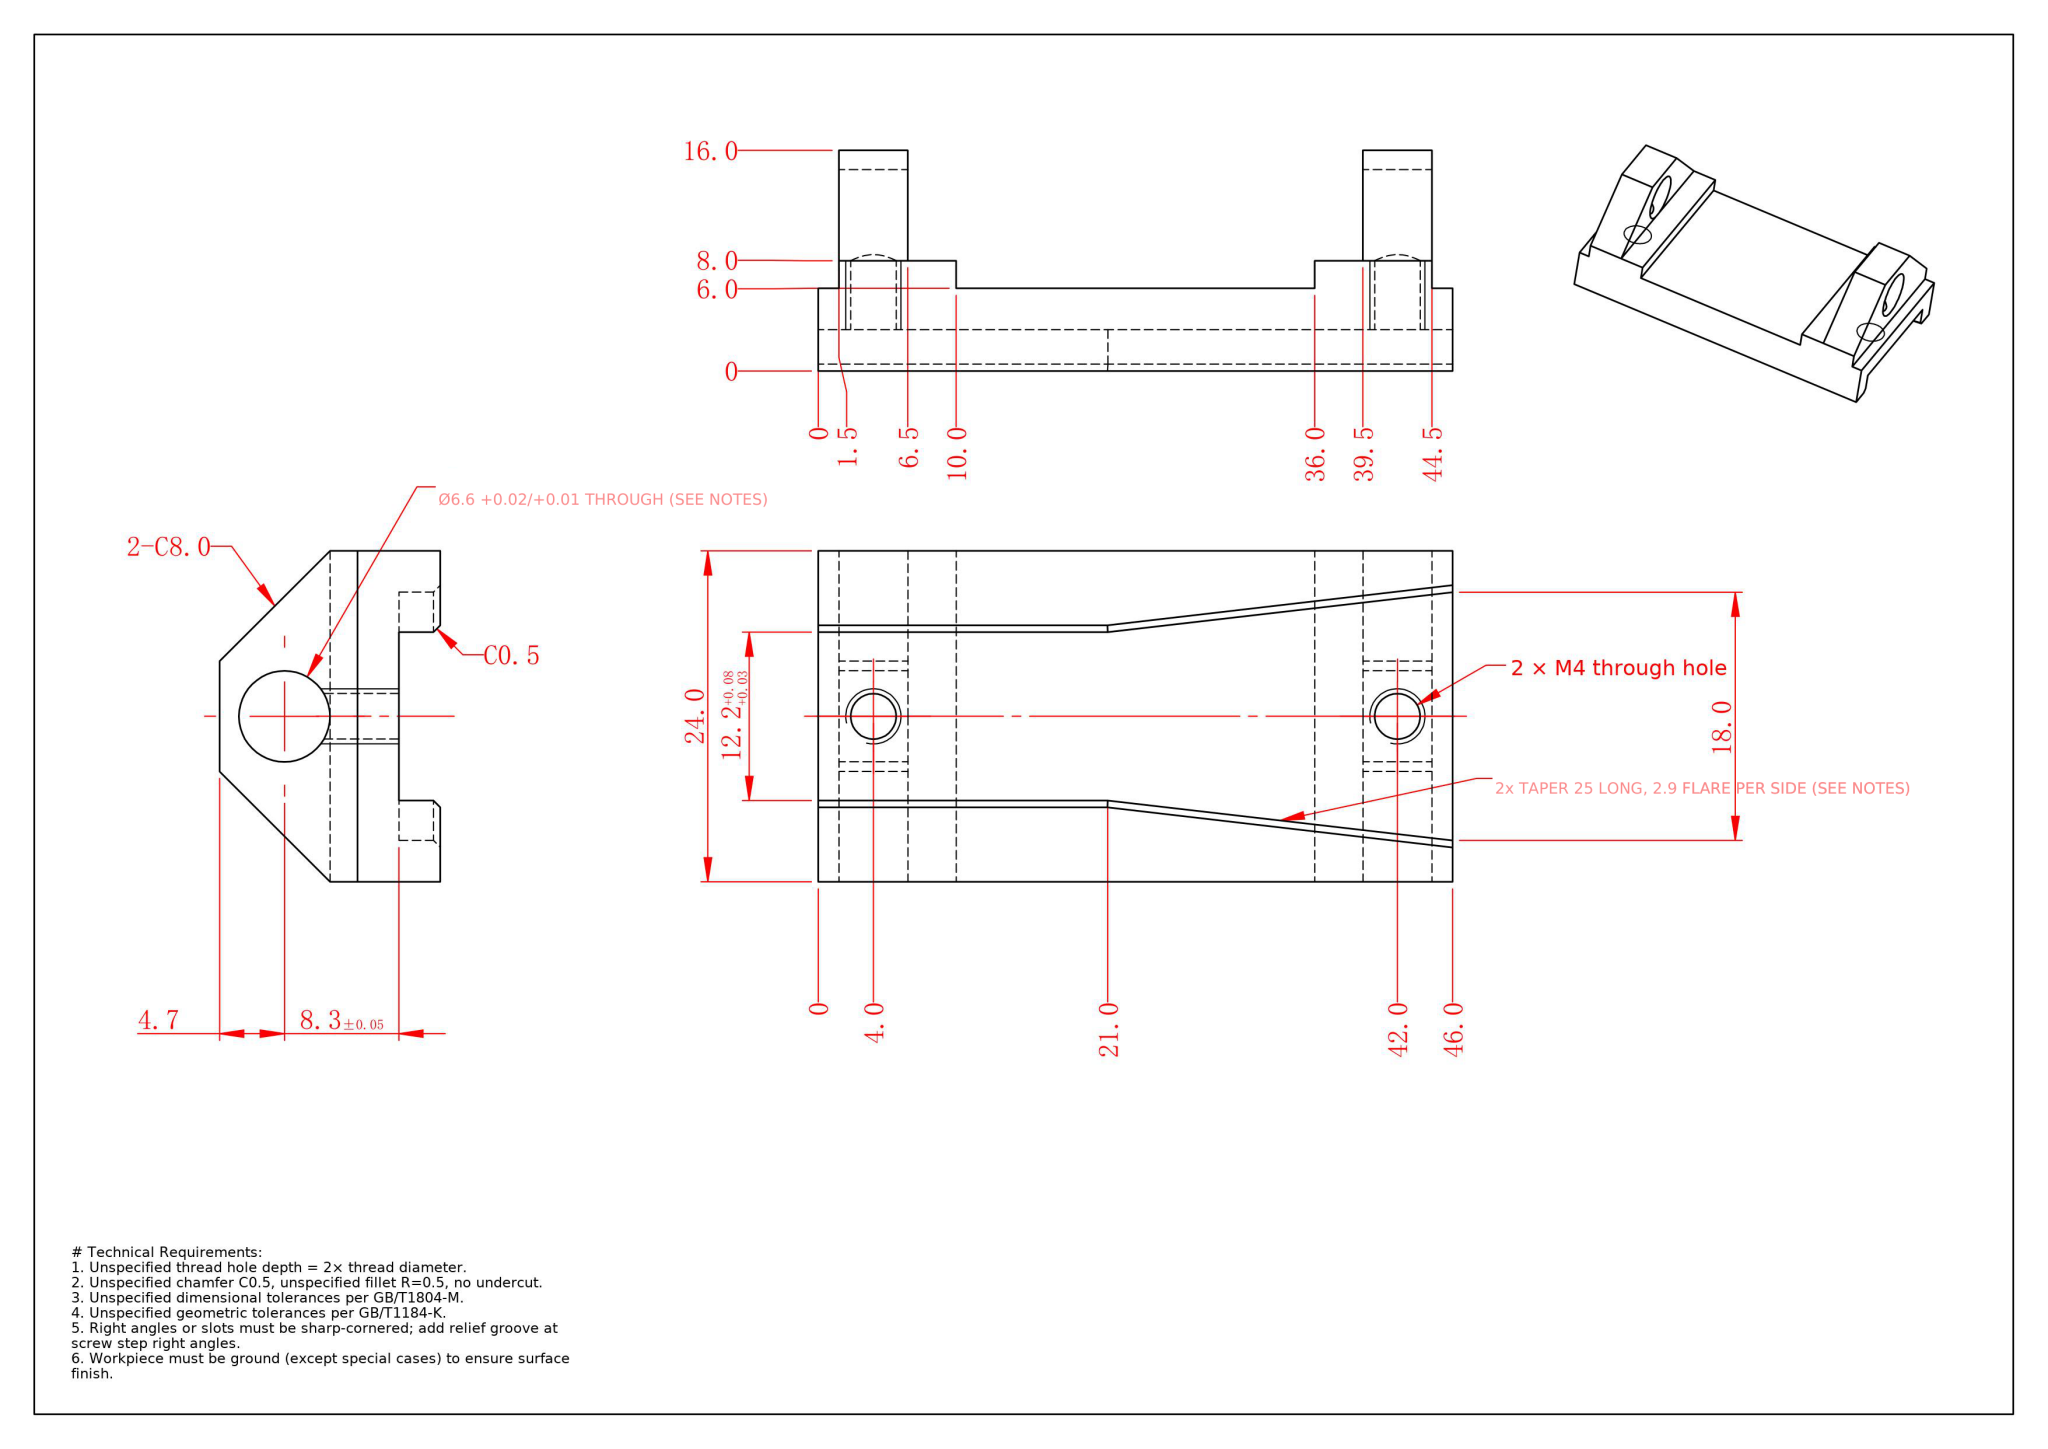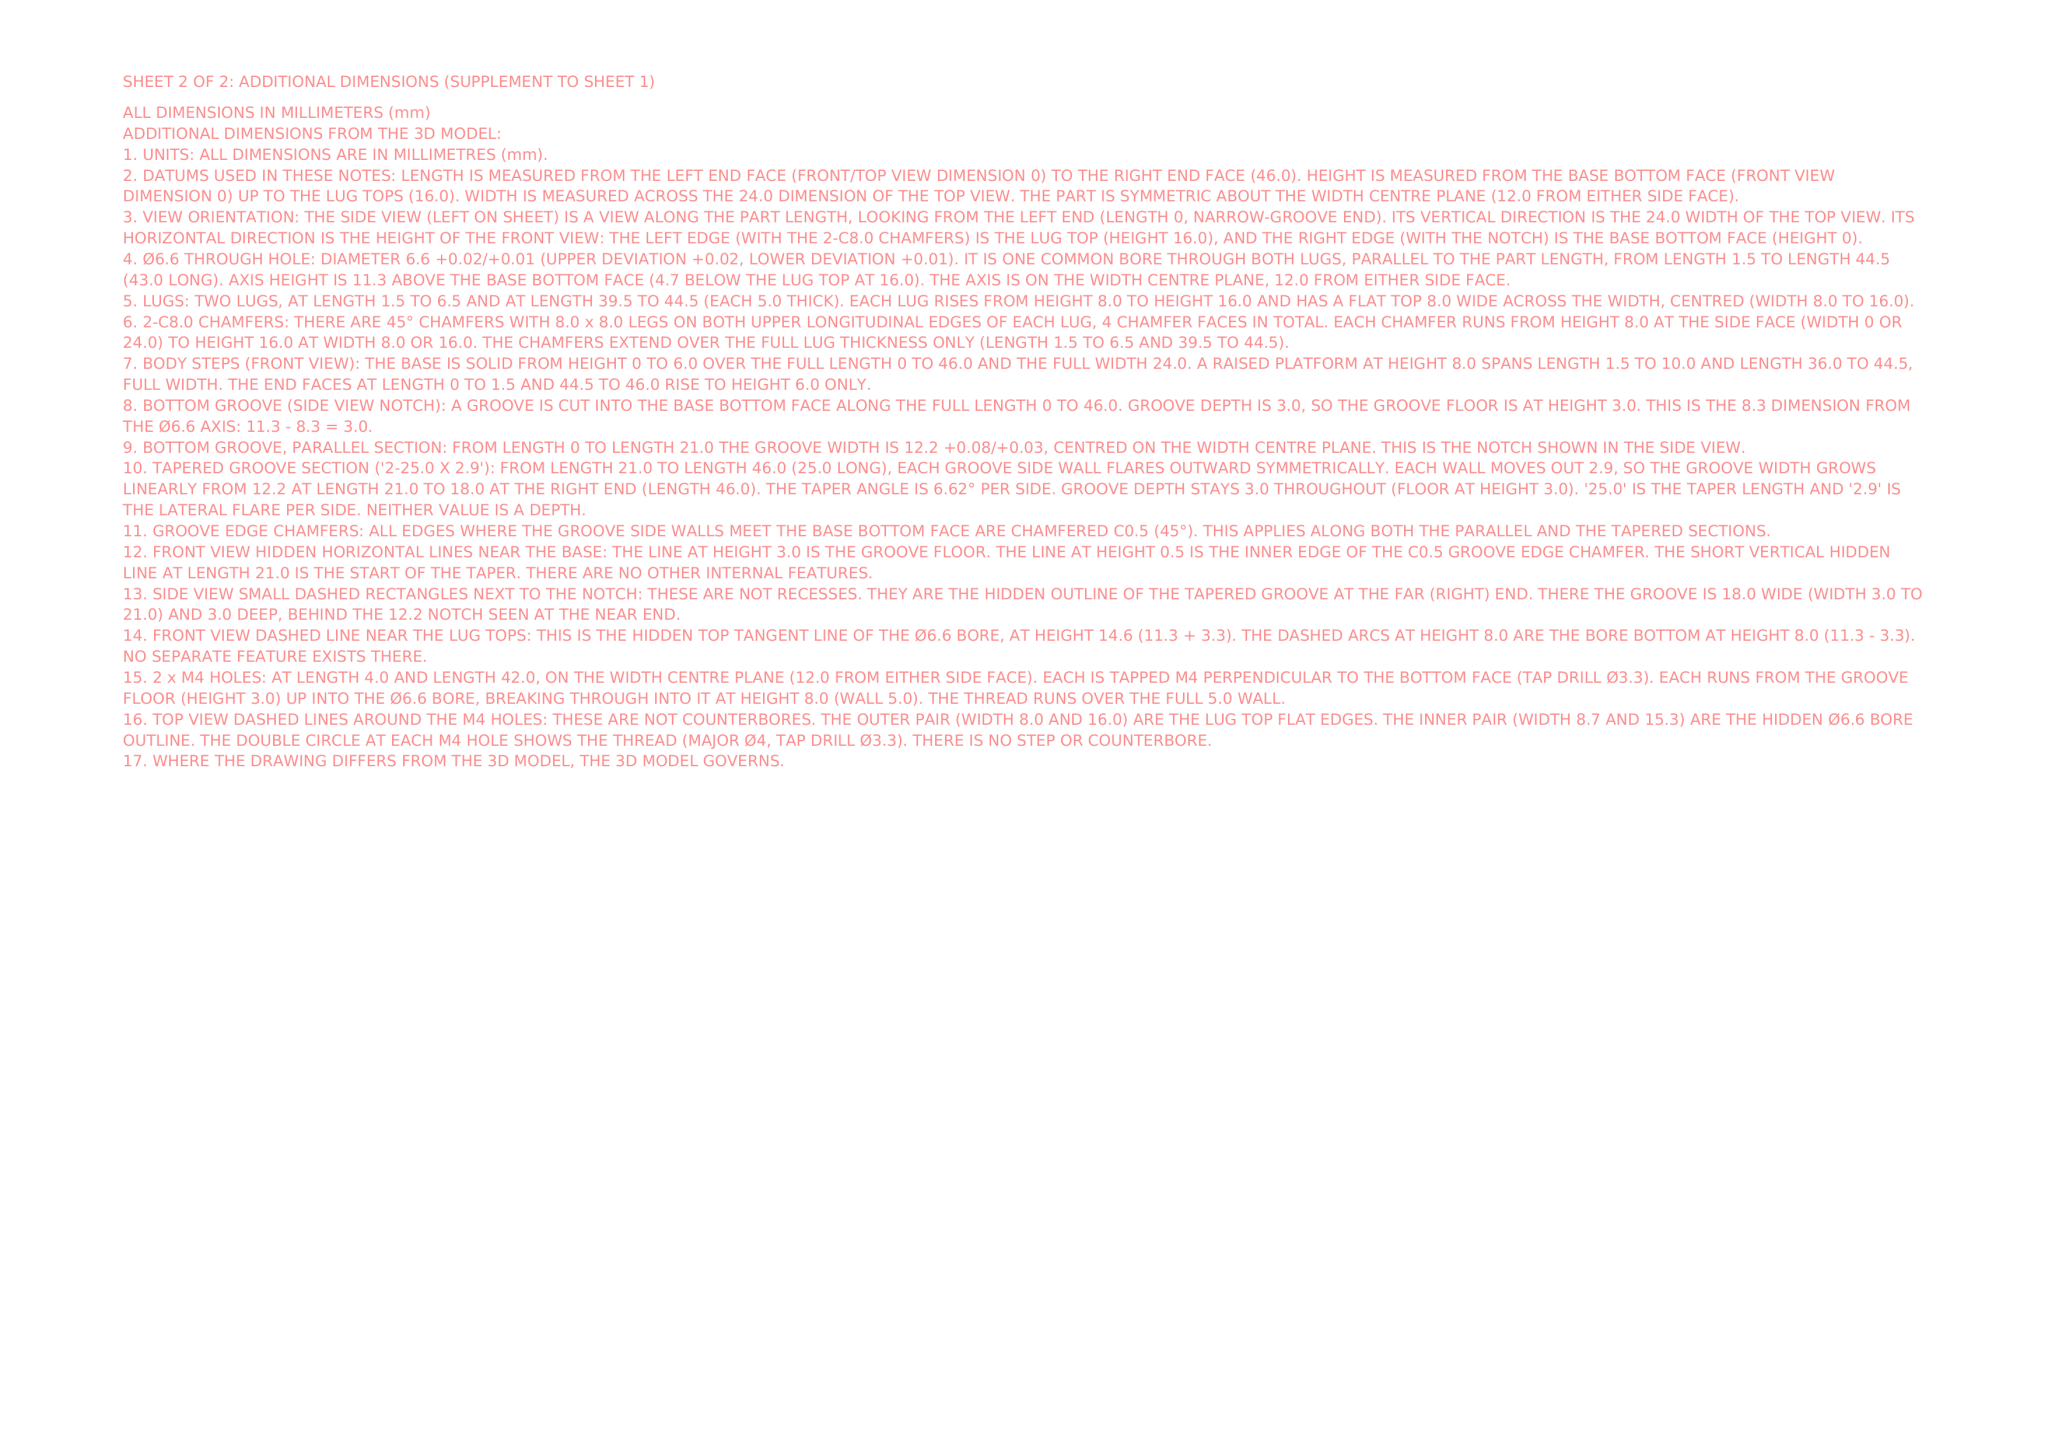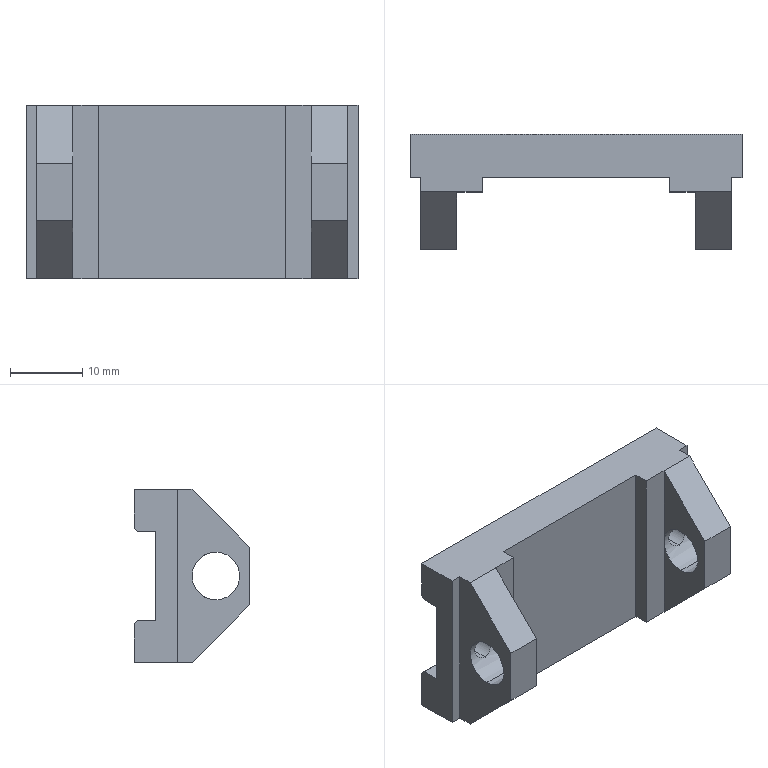Part | NX | mm | Stepped Angled Rail Bracket | 1 solid | 40 faces | box 46 x 16 x 24 mm | volume 6378 mm3 | plane 32 | cylinder 8 | commonest cylinder face diameters 3.3 x4 6.6 x4